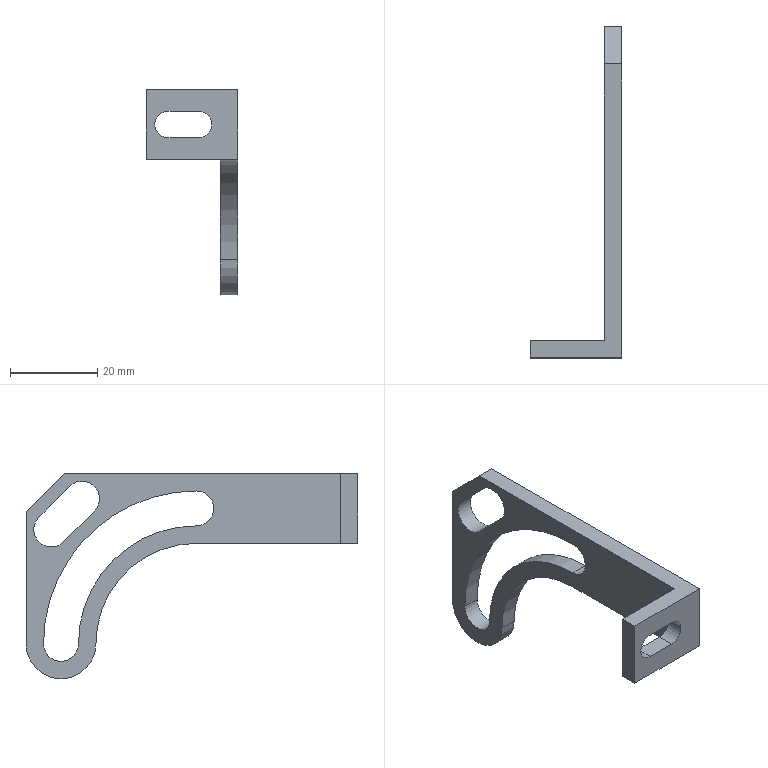Component | NX | BRACKET | 1 solid | 23 faces | volume 5567 mm3 | plane 13 | cylinder 10 | commonest cylinder face diameters 8 x4 6 x2 54 x1 16 x1 46 x1 70 x1